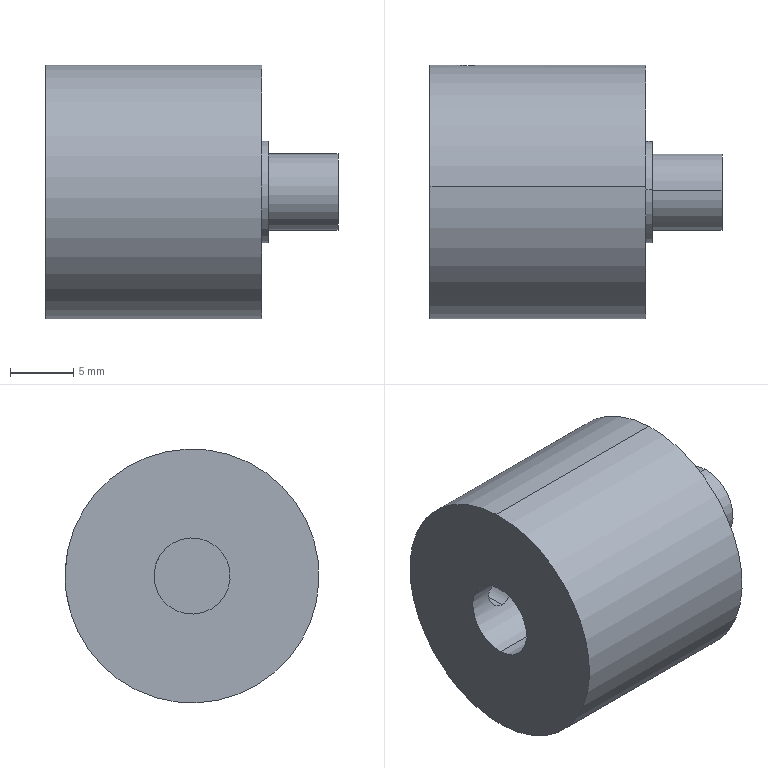Component | SolidWorks | AS-011-JG0108-1 | 1 solid | 15 faces | box 23 x 20 x 20 mm | volume 5133 mm3 | cylinder 10 | plane 5 | commonest cylinder face diameters 6 x4 2.5 x2 20 x2 8 x2
build123d program:
from build123d import *

# Parameters (mm, degrees)
SKETCH2_R          = 1.25
CUT_EXTRUDE1_DEPTH = 22
CUT_EXTRUDE2_START = -36
SKETCH3_R          = 15
SKETCH3_R_2        = 10
CUT_EXTRUDE2_DEPTH = 36


with BuildPart() as part:
    # Sketch1 → Revolve1 (revolve)
    with BuildSketch(Plane.XY, mode=Mode.PRIVATE) as revolve1_sk:
        Polygon((-6, 15), (-23, 15), (-23, 3), (-10.5, 3), (-10.5, 0), (0, 0), (0, 3), (-5.5, 3), (-5.5, 4), (-6, 4), align=None)
    revolve(revolve1_sk.sketch.rotate(Axis((-10.5, 0, 0), (1, 0, 0)), 90), axis=Axis((-10.5, 0, 0), (1, 0, 0)))

    # Sketch2 → Cut-Extrude1 (cut)
    with BuildSketch(Plane(origin=(0, 0, 0), x_dir=(1, 0, 0), z_dir=(0, 1, 0))):
        with Locations(Location((-20, 0, 0), (0, 0, 270))):
            Circle(SKETCH2_R)
    extrude(amount=-CUT_EXTRUDE1_DEPTH, mode=Mode.SUBTRACT)

    # Sketch3 → Cut-Extrude2 (cut)
    with BuildSketch(Plane(origin=(-6, 0, 0), x_dir=(0, 0, -1), z_dir=(1, 0, 0)).offset(CUT_EXTRUDE2_START)):
        Circle(SKETCH3_R)
        Circle(SKETCH3_R_2, mode=Mode.SUBTRACT)
    extrude(amount=CUT_EXTRUDE2_DEPTH, mode=Mode.SUBTRACT)


solid = part.part

# Placed as in the assembly
solid = solid.moved(Location((-0.5, -18, -10), (177.746, 0, 0.001754)))
STEP:
#1=CARTESIAN_POINT('',(-0.8071,-0.3164,-0.3598));
#2=VERTEX_POINT('',#1);
#3=CARTESIAN_POINT('',(-0.8071,-0.3203,-0.4582));
#4=VERTEX_POINT('',#3);
#5=CARTESIAN_POINT('',(-0.8071,-0.3164,-0.3598));
#6=CARTESIAN_POINT('',(-0.8135,-0.3164,-0.3598));
#7=CARTESIAN_POINT('',(-0.82,-0.3163,-0.3611));
#8=CARTESIAN_POINT('',(-0.8318,-0.3159,-0.366));
#9=CARTESIAN_POINT('',(-0.8373,-0.3157,-0.3697));
#10=CARTESIAN_POINT('',(-0.8464,-0.3152,-0.3788));
#11=CARTESIAN_POINT('',(-0.8501,-0.315,-0.3843));
#12=CARTESIAN_POINT('',(-0.855,-0.3149,-0.3962));
#13=CARTESIAN_POINT('',(-0.8563,-0.315,-0.4026));
#14=CARTESIAN_POINT('',(-0.8563,-0.3155,-0.4156));
#15=CARTESIAN_POINT('',(-0.855,-0.3159,-0.422));
#16=CARTESIAN_POINT('',(-0.8501,-0.317,-0.4338));
#17=CARTESIAN_POINT('',(-0.8464,-0.3176,-0.4393));
#18=CARTESIAN_POINT('',(-0.8374,-0.3187,-0.4483));
#19=CARTESIAN_POINT('',(-0.8319,-0.3193,-0.452));
#20=CARTESIAN_POINT('',(-0.8201,-0.3201,-0.4569));
#21=CARTESIAN_POINT('',(-0.8136,-0.3203,-0.4582));
#22=CARTESIAN_POINT('',(-0.8071,-0.3203,-0.4582));
#23=B_SPLINE_CURVE_WITH_KNOTS('',3,(#5,#6,#7,#8,#9,#10,#11,#12,#13,#14,#15,#16,#17,#18,#19,#20,#21,#22),.UNSPECIFIED.,.F.,.F.,(4,2,2,2,2,2,2,2,4),(0.003912,0.004401,0.00489,0.005379,0.005867,0.006356,0.006845,0.007334,0.007823),.UNSPECIFIED.);
#24=EDGE_CURVE('',#2,#4,#23,.T.);
#25=ORIENTED_EDGE('',*,*,#24,.F.);
#26=CARTESIAN_POINT('',(-0.8071,-0.5994,-0.3487));
#27=VERTEX_POINT('',#26);
#28=CARTESIAN_POINT('',(-0.8071,0.1587,-0.3784));
#29=DIRECTION('',(0.,-0.9992,0.03916));
#30=VECTOR('',#29,39.37);
#31=LINE('',#28,#30);
#32=EDGE_CURVE('',#2,#27,#31,.T.);
#33=ORIENTED_EDGE('',*,*,#32,.T.);
#34=CARTESIAN_POINT('',(-0.8071,-0.6033,-0.4471));
#35=VERTEX_POINT('',#34);
#36=CARTESIAN_POINT('',(-0.8071,-0.6033,-0.4471));
#37=CARTESIAN_POINT('',(-0.8104,-0.6033,-0.4471));
#38=CARTESIAN_POINT('',(-0.8136,-0.6031,-0.4468));
#39=CARTESIAN_POINT('',(-0.8199,-0.6025,-0.4455));
#40=CARTESIAN_POINT('',(-0.8231,-0.6021,-0.4446));
#41=CARTESIAN_POINT('',(-0.832,-0.6004,-0.4409));
#42=CARTESIAN_POINT('',(-0.8374,-0.5988,-0.4373));
#43=CARTESIAN_POINT('',(-0.8464,-0.5957,-0.4285));
#44=CARTESIAN_POINT('',(-0.85,-0.5941,-0.4231));
#45=CARTESIAN_POINT('',(-0.855,-0.5917,-0.4114));
#46=CARTESIAN_POINT('',(-0.8563,-0.5909,-0.4049));
#47=CARTESIAN_POINT('',(-0.8563,-0.5905,-0.3951));
#48=CARTESIAN_POINT('',(-0.856,-0.5905,-0.3918));
#49=CARTESIAN_POINT('',(-0.8547,-0.5908,-0.3854));
#50=CARTESIAN_POINT('',(-0.8537,-0.5911,-0.3823));
#51=CARTESIAN_POINT('',(-0.85,-0.5922,-0.3733));
#52=CARTESIAN_POINT('',(-0.8464,-0.5933,-0.3679));
#53=CARTESIAN_POINT('',(-0.8373,-0.5957,-0.3588));
#54=CARTESIAN_POINT('',(-0.8319,-0.597,-0.3551));
#55=CARTESIAN_POINT('',(-0.8201,-0.5989,-0.3501));
#56=CARTESIAN_POINT('',(-0.8136,-0.5994,-0.3487));
#57=CARTESIAN_POINT('',(-0.8071,-0.5994,-0.3487));
#58=B_SPLINE_CURVE_WITH_KNOTS('',3,(#36,#37,#38,#39,#40,#41,#42,#43,#44,#45,#46,#47,#48,#49,#50,#51,#52,#53,#54,#55,#56,#57),.UNSPECIFIED.,.F.,.F.,(4,2,2,2,2,2,2,2,2,2,4),(0.,0.0002471,0.0004942,0.0009884,0.001483,0.001977,0.002224,0.002471,0.002965,0.003459,0.003953),.UNSPECIFIED.);
#59=EDGE_CURVE('',#35,#27,#58,.T.);
#60=ORIENTED_EDGE('',*,*,#59,.F.);
#61=CARTESIAN_POINT('',(-0.8071,0.1549,-0.4768));
#62=DIRECTION('',(0.,-0.9992,0.03916));
#63=VECTOR('',#62,39.37);
#64=LINE('',#61,#63);
#65=EDGE_CURVE('',#4,#35,#64,.T.);
#66=ORIENTED_EDGE('',*,*,#65,.F.);
#67=EDGE_LOOP('',(#25,#33,#60,#66));
#68=FACE_OUTER_BOUND('',#67,.T.);
#69=CARTESIAN_POINT('',(-0.8071,0.1568,-0.4276));
#70=DIRECTION('',(0.,-0.9992,0.03916));
#71=DIRECTION('',(0.,-0.03916,-0.9992));
#72=AXIS2_PLACEMENT_3D('',#69,#70,#71);
#73=CYLINDRICAL_SURFACE('',#72,0.04921);
#74=ADVANCED_FACE('',(#68),#73,.F.);
#75=ORIENTED_EDGE('',*,*,#59,.T.);
#76=CARTESIAN_POINT('',(-0.8071,-0.5994,-0.3487));
#77=CARTESIAN_POINT('',(-0.8006,-0.5994,-0.3487));
#78=CARTESIAN_POINT('',(-0.7941,-0.5989,-0.3501));
#79=CARTESIAN_POINT('',(-0.7822,-0.597,-0.3551));
#80=CARTESIAN_POINT('',(-0.7768,-0.5957,-0.3588));
#81=CARTESIAN_POINT('',(-0.77,-0.5939,-0.3656));
#82=CARTESIAN_POINT('',(-0.768,-0.5933,-0.3681));
#83=CARTESIAN_POINT('',(-0.7645,-0.5923,-0.3735));
#84=CARTESIAN_POINT('',(-0.7629,-0.5918,-0.3763));
#85=CARTESIAN_POINT('',(-0.7604,-0.5911,-0.3823));
#86=CARTESIAN_POINT('',(-0.7595,-0.5908,-0.3854));
#87=CARTESIAN_POINT('',(-0.7582,-0.5905,-0.3918));
#88=CARTESIAN_POINT('',(-0.7579,-0.5905,-0.3951));
#89=CARTESIAN_POINT('',(-0.7579,-0.5909,-0.4048));
#90=CARTESIAN_POINT('',(-0.7592,-0.5917,-0.4113));
#91=CARTESIAN_POINT('',(-0.7641,-0.5941,-0.4231));
#92=CARTESIAN_POINT('',(-0.7678,-0.5957,-0.4284));
#93=CARTESIAN_POINT('',(-0.7768,-0.5988,-0.4374));
#94=CARTESIAN_POINT('',(-0.7821,-0.6004,-0.4409));
#95=CARTESIAN_POINT('',(-0.7941,-0.6026,-0.4458));
#96=CARTESIAN_POINT('',(-0.8005,-0.6033,-0.4471));
#97=CARTESIAN_POINT('',(-0.8071,-0.6033,-0.4471));
#98=B_SPLINE_CURVE_WITH_KNOTS('',3,(#76,#77,#78,#79,#80,#81,#82,#83,#84,#85,#86,#87,#88,#89,#90,#91,#92,#93,#94,#95,#96,#97),.UNSPECIFIED.,.F.,.F.,(4,2,2,2,2,2,2,2,2,2,4),(0.003953,0.004447,0.004941,0.005188,0.005435,0.005682,0.005929,0.006422,0.006916,0.00741,0.007904),.UNSPECIFIED.);
#99=EDGE_CURVE('',#27,#35,#98,.T.);
#100=ORIENTED_EDGE('',*,*,#99,.T.);
#101=EDGE_LOOP('',(#75,#100));
#102=FACE_BOUND('',#101,.T.);
#103=CARTESIAN_POINT('',(-0.4331,-0.704,-0.2757));
#104=VERTEX_POINT('',#103);
#105=CARTESIAN_POINT('',(-0.4331,-0.7133,-0.5117));
#106=VERTEX_POINT('',#105);
#107=CARTESIAN_POINT('',(-0.4331,-0.7087,-0.3937));
#108=DIRECTION('',(-1.,0.,0.));
#109=DIRECTION('',(0.,-0.03916,-0.9992));
#110=AXIS2_PLACEMENT_3D('',#107,#108,#109);
#111=CIRCLE('',#110,0.1181);
#112=EDGE_CURVE('',#104,#106,#111,.T.);
#113=ORIENTED_EDGE('',*,*,#112,.F.);
#114=CARTESIAN_POINT('',(-0.9252,-0.704,-0.2757));
#115=VERTEX_POINT('',#114);
#116=CARTESIAN_POINT('',(-0.4331,-0.704,-0.2757));
#117=DIRECTION('',(-1.,0.,0.));
#118=VECTOR('',#117,39.37);
#119=LINE('',#116,#118);
#120=EDGE_CURVE('',#104,#115,#119,.T.);
#121=ORIENTED_EDGE('',*,*,#120,.T.);
#122=CARTESIAN_POINT('',(-0.9252,-0.7133,-0.5117));
#123=VERTEX_POINT('',#122);
#124=CARTESIAN_POINT('',(-0.9252,-0.7087,-0.3937));
#125=DIRECTION('',(-1.,0.,0.));
#126=DIRECTION('',(0.,-0.03916,-0.9992));
#127=AXIS2_PLACEMENT_3D('',#124,#125,#126);
#128=CIRCLE('',#127,0.1181);
#129=EDGE_CURVE('',#115,#123,#128,.T.);
#130=ORIENTED_EDGE('',*,*,#129,.T.);
#131=CARTESIAN_POINT('',(-0.4331,-0.7133,-0.5117));
#132=DIRECTION('',(-1.,0.,0.));
#133=VECTOR('',#132,39.37);
#134=LINE('',#131,#133);
#135=EDGE_CURVE('',#106,#123,#134,.T.);
#136=ORIENTED_EDGE('',*,*,#135,.F.);
#137=EDGE_LOOP('',(#113,#121,#130,#136));
#138=FACE_OUTER_BOUND('',#137,.T.);
#139=CARTESIAN_POINT('',(-0.4331,-0.7087,-0.3937));
#140=DIRECTION('',(-1.,0.,0.));
#141=DIRECTION('',(0.,-0.03916,-0.9992));
#142=AXIS2_PLACEMENT_3D('',#139,#140,#141);
#143=CYLINDRICAL_SURFACE('',#142,0.1181);
#144=ADVANCED_FACE('',(#102,#138),#143,.F.);
#145=CARTESIAN_POINT('',(-0.9252,-0.6932,-0.000302));
#146=VERTEX_POINT('',#145);
#147=CARTESIAN_POINT('',(-0.9252,-0.7241,-0.7871));
#148=VERTEX_POINT('',#147);
#149=CARTESIAN_POINT('',(-0.9252,-0.7087,-0.3937));
#150=DIRECTION('',(1.,0.,0.));
#151=DIRECTION('',(0.,0.03916,0.9992));
#152=AXIS2_PLACEMENT_3D('',#149,#150,#151);
#153=CIRCLE('',#152,0.3937);
#154=EDGE_CURVE('',#146,#148,#153,.T.);
#155=ORIENTED_EDGE('',*,*,#154,.T.);
#156=CARTESIAN_POINT('',(-0.2559,-0.7241,-0.7871));
#157=VERTEX_POINT('',#156);
#158=CARTESIAN_POINT('',(-1.673,-0.7241,-0.7871));
#159=DIRECTION('',(1.,0.,0.));
#160=VECTOR('',#159,39.37);
#161=LINE('',#158,#160);
#162=EDGE_CURVE('',#148,#157,#161,.T.);
#163=ORIENTED_EDGE('',*,*,#162,.T.);
#164=CARTESIAN_POINT('',(-0.2559,-0.6932,-0.000302));
#165=VERTEX_POINT('',#164);
#166=CARTESIAN_POINT('',(-0.2559,-0.7087,-0.3937));
#167=DIRECTION('',(1.,0.,0.));
#168=DIRECTION('',(0.,0.03916,0.9992));
#169=AXIS2_PLACEMENT_3D('',#166,#167,#168);
#170=CIRCLE('',#169,0.3937);
#171=EDGE_CURVE('',#165,#157,#170,.T.);
#172=ORIENTED_EDGE('',*,*,#171,.F.);
#173=CARTESIAN_POINT('',(-1.673,-0.6932,-0.000302));
#174=DIRECTION('',(1.,0.,0.));
#175=VECTOR('',#174,39.37);
#176=LINE('',#173,#175);
#177=EDGE_CURVE('',#146,#165,#176,.T.);
#178=ORIENTED_EDGE('',*,*,#177,.F.);
#179=EDGE_LOOP('',(#155,#163,#172,#178));
#180=FACE_OUTER_BOUND('',#179,.T.);
#181=CARTESIAN_POINT('',(-1.673,-0.7087,-0.3937));
#182=DIRECTION('',(1.,0.,0.));
#183=DIRECTION('',(0.,0.03916,0.9992));
#184=AXIS2_PLACEMENT_3D('',#181,#182,#183);
#185=CYLINDRICAL_SURFACE('',#184,0.3937);
#186=ADVANCED_FACE('',(#180),#185,.T.);
#187=CARTESIAN_POINT('',(-0.01969,-0.7133,-0.5117));
#188=VERTEX_POINT('',#187);
#189=CARTESIAN_POINT('',(-0.01969,-0.704,-0.2757));
#190=VERTEX_POINT('',#189);
#191=CARTESIAN_POINT('',(-0.01969,-0.7087,-0.3937));
#192=DIRECTION('',(-1.,0.,0.));
#193=DIRECTION('',(0.,-0.03916,-0.9992));
#194=AXIS2_PLACEMENT_3D('',#191,#192,#193);
#195=CIRCLE('',#194,0.1181);
#196=EDGE_CURVE('',#188,#190,#195,.T.);
#197=ORIENTED_EDGE('',*,*,#196,.T.);
#198=CARTESIAN_POINT('',(-0.2362,-0.704,-0.2757));
#199=VERTEX_POINT('',#198);
#200=CARTESIAN_POINT('',(-0.4331,-0.704,-0.2757));
#201=DIRECTION('',(-1.,0.,0.));
#202=VECTOR('',#201,39.37);
#203=LINE('',#200,#202);
#204=EDGE_CURVE('',#190,#199,#203,.T.);
#205=ORIENTED_EDGE('',*,*,#204,.T.);
#206=CARTESIAN_POINT('',(-0.2362,-0.7133,-0.5117));
#207=VERTEX_POINT('',#206);
#208=CARTESIAN_POINT('',(-0.2362,-0.7087,-0.3937));
#209=DIRECTION('',(-1.,0.,0.));
#210=DIRECTION('',(0.,-0.03916,-0.9992));
#211=AXIS2_PLACEMENT_3D('',#208,#209,#210);
#212=CIRCLE('',#211,0.1181);
#213=EDGE_CURVE('',#207,#199,#212,.T.);
#214=ORIENTED_EDGE('',*,*,#213,.F.);
#215=CARTESIAN_POINT('',(-0.4331,-0.7133,-0.5117));
#216=DIRECTION('',(-1.,0.,0.));
#217=VECTOR('',#216,39.37);
#218=LINE('',#215,#217);
#219=EDGE_CURVE('',#188,#207,#218,.T.);
#220=ORIENTED_EDGE('',*,*,#219,.F.);
#221=EDGE_LOOP('',(#197,#205,#214,#220));
#222=FACE_OUTER_BOUND('',#221,.T.);
#223=CARTESIAN_POINT('',(-0.4331,-0.7087,-0.3937));
#224=DIRECTION('',(-1.,0.,0.));
#225=DIRECTION('',(0.,-0.03916,-0.9992));
#226=AXIS2_PLACEMENT_3D('',#223,#224,#225);
#227=CYLINDRICAL_SURFACE('',#226,0.1181);
#228=ADVANCED_FACE('',(#222),#227,.T.);
#229=CARTESIAN_POINT('',(-0.2362,-0.7148,-0.5511));
#230=VERTEX_POINT('',#229);
#231=CARTESIAN_POINT('',(-0.2362,-0.7025,-0.2363));
#232=VERTEX_POINT('',#231);
#233=CARTESIAN_POINT('',(-0.2362,-0.7087,-0.3937));
#234=DIRECTION('',(-1.,0.,0.));
#235=DIRECTION('',(0.,-0.03916,-0.9992));
#236=AXIS2_PLACEMENT_3D('',#233,#234,#235);
#237=CIRCLE('',#236,0.1575);
#238=EDGE_CURVE('',#230,#232,#237,.T.);
#239=ORIENTED_EDGE('',*,*,#238,.T.);
#240=CARTESIAN_POINT('',(-0.2559,-0.7025,-0.2363));
#241=VERTEX_POINT('',#240);
#242=CARTESIAN_POINT('',(-0.4331,-0.7025,-0.2363));
#243=DIRECTION('',(-1.,0.,0.));
#244=VECTOR('',#243,39.37);
#245=LINE('',#242,#244);
#246=EDGE_CURVE('',#232,#241,#245,.T.);
#247=ORIENTED_EDGE('',*,*,#246,.T.);
#248=CARTESIAN_POINT('',(-0.2559,-0.7148,-0.5511));
#249=VERTEX_POINT('',#248);
#250=CARTESIAN_POINT('',(-0.2559,-0.7087,-0.3937));
#251=DIRECTION('',(-1.,0.,0.));
#252=DIRECTION('',(0.,-0.03916,-0.9992));
#253=AXIS2_PLACEMENT_3D('',#250,#251,#252);
#254=CIRCLE('',#253,0.1575);
#255=EDGE_CURVE('',#249,#241,#254,.T.);
#256=ORIENTED_EDGE('',*,*,#255,.F.);
#257=CARTESIAN_POINT('',(-0.4331,-0.7148,-0.5511));
#258=DIRECTION('',(-1.,0.,0.));
#259=VECTOR('',#258,39.37);
#260=LINE('',#257,#259);
#261=EDGE_CURVE('',#230,#249,#260,.T.);
#262=ORIENTED_EDGE('',*,*,#261,.F.);
#263=EDGE_LOOP('',(#239,#247,#256,#262));
#264=FACE_OUTER_BOUND('',#263,.T.);
#265=CARTESIAN_POINT('',(-0.4331,-0.7087,-0.3937));
#266=DIRECTION('',(-1.,0.,0.));
#267=DIRECTION('',(0.,-0.03916,-0.9992));
#268=AXIS2_PLACEMENT_3D('',#265,#266,#267);
#269=CYLINDRICAL_SURFACE('',#268,0.1575);
#270=ADVANCED_FACE('',(#264),#269,.T.);
#271=ORIENTED_EDGE('',*,*,#255,.T.);
#272=CARTESIAN_POINT('',(-0.2559,-0.7087,-0.3937));
#273=DIRECTION('',(-1.,0.,0.));
#274=DIRECTION('',(0.,-0.03916,-0.9992));
#275=AXIS2_PLACEMENT_3D('',#272,#273,#274);
#276=CIRCLE('',#275,0.1575);
#277=EDGE_CURVE('',#241,#249,#276,.T.);
#278=ORIENTED_EDGE('',*,*,#277,.T.);
#279=EDGE_LOOP('',(#271,#278));
#280=FACE_BOUND('',#279,.T.);
#281=ORIENTED_EDGE('',*,*,#171,.T.);
#282=CARTESIAN_POINT('',(-0.2559,-0.7087,-0.3937));
#283=DIRECTION('',(1.,0.,0.));
#284=DIRECTION('',(0.,0.03916,0.9992));
#285=AXIS2_PLACEMENT_3D('',#282,#283,#284);
#286=CIRCLE('',#285,0.3937);
#287=EDGE_CURVE('',#157,#165,#286,.T.);
#288=ORIENTED_EDGE('',*,*,#287,.T.);
#289=EDGE_LOOP('',(#281,#288));
#290=FACE_OUTER_BOUND('',#289,.T.);
#291=CARTESIAN_POINT('',(-0.2559,-1.299,-0.3706));
#292=DIRECTION('',(-1.,0.,0.));
#293=DIRECTION('',(0.,-0.03916,-0.9992));
#294=AXIS2_PLACEMENT_3D('',#291,#292,#293);
#295=PLANE('',#294);
#296=ADVANCED_FACE('',(#280,#290),#295,.F.);
#297=ORIENTED_EDGE('',*,*,#246,.F.);
#298=CARTESIAN_POINT('',(-0.2362,-0.7087,-0.3937));
#299=DIRECTION('',(-1.,0.,0.));
#300=DIRECTION('',(0.,-0.03916,-0.9992));
#301=AXIS2_PLACEMENT_3D('',#298,#299,#300);
#302=CIRCLE('',#301,0.1575);
#303=EDGE_CURVE('',#232,#230,#302,.T.);
#304=ORIENTED_EDGE('',*,*,#303,.T.);
#305=ORIENTED_EDGE('',*,*,#261,.T.);
#306=ORIENTED_EDGE('',*,*,#277,.F.);
#307=EDGE_LOOP('',(#297,#304,#305,#306));
#308=FACE_OUTER_BOUND('',#307,.T.);
#309=CARTESIAN_POINT('',(-0.4331,-0.7087,-0.3937));
#310=DIRECTION('',(-1.,0.,0.));
#311=DIRECTION('',(0.,-0.03916,-0.9992));
#312=AXIS2_PLACEMENT_3D('',#309,#310,#311);
#313=CYLINDRICAL_SURFACE('',#312,0.1575);
#314=ADVANCED_FACE('',(#308),#313,.T.);
#315=ORIENTED_EDGE('',*,*,#238,.F.);
#316=ORIENTED_EDGE('',*,*,#303,.F.);
#317=EDGE_LOOP('',(#315,#316));
#318=FACE_OUTER_BOUND('',#317,.T.);
#319=ORIENTED_EDGE('',*,*,#213,.T.);
#320=CARTESIAN_POINT('',(-0.2362,-0.7087,-0.3937));
#321=DIRECTION('',(-1.,0.,0.));
#322=DIRECTION('',(0.,-0.03916,-0.9992));
#323=AXIS2_PLACEMENT_3D('',#320,#321,#322);
#324=CIRCLE('',#323,0.1181);
#325=EDGE_CURVE('',#199,#207,#324,.T.);
#326=ORIENTED_EDGE('',*,*,#325,.T.);
#327=EDGE_LOOP('',(#319,#326));
#328=FACE_BOUND('',#327,.T.);
#329=CARTESIAN_POINT('',(-0.2362,-0.866,-0.3875));
#330=DIRECTION('',(-1.,0.,0.));
#331=DIRECTION('',(0.,-0.03916,-0.9992));
#332=AXIS2_PLACEMENT_3D('',#329,#330,#331);
#333=PLANE('',#332);
#334=ADVANCED_FACE('',(#318,#328),#333,.F.);
#335=ORIENTED_EDGE('',*,*,#204,.F.);
#336=CARTESIAN_POINT('',(-0.01969,-0.7087,-0.3937));
#337=DIRECTION('',(-1.,0.,0.));
#338=DIRECTION('',(0.,-0.03916,-0.9992));
#339=AXIS2_PLACEMENT_3D('',#336,#337,#338);
#340=CIRCLE('',#339,0.1181);
#341=EDGE_CURVE('',#190,#188,#340,.T.);
#342=ORIENTED_EDGE('',*,*,#341,.T.);
#343=ORIENTED_EDGE('',*,*,#219,.T.);
#344=ORIENTED_EDGE('',*,*,#325,.F.);
#345=EDGE_LOOP('',(#335,#342,#343,#344));
#346=FACE_OUTER_BOUND('',#345,.T.);
#347=CARTESIAN_POINT('',(-0.4331,-0.7087,-0.3937));
#348=DIRECTION('',(-1.,0.,0.));
#349=DIRECTION('',(0.,-0.03916,-0.9992));
#350=AXIS2_PLACEMENT_3D('',#347,#348,#349);
#351=CYLINDRICAL_SURFACE('',#350,0.1181);
#352=ADVANCED_FACE('',(#346),#351,.T.);
#353=ORIENTED_EDGE('',*,*,#196,.F.);
#354=ORIENTED_EDGE('',*,*,#341,.F.);
#355=EDGE_LOOP('',(#353,#354));
#356=FACE_OUTER_BOUND('',#355,.T.);
#357=CARTESIAN_POINT('',(-0.01969,-0.8267,-0.3891));
#358=DIRECTION('',(-1.,0.,0.));
#359=DIRECTION('',(0.,-0.03916,-0.9992));
#360=AXIS2_PLACEMENT_3D('',#357,#358,#359);
#361=PLANE('',#360);
#362=ADVANCED_FACE('',(#356),#361,.F.);
#363=ORIENTED_EDGE('',*,*,#162,.F.);
#364=CARTESIAN_POINT('',(-0.9252,-0.7087,-0.3937));
#365=DIRECTION('',(1.,0.,0.));
#366=DIRECTION('',(0.,0.03916,0.9992));
#367=AXIS2_PLACEMENT_3D('',#364,#365,#366);
#368=CIRCLE('',#367,0.3937);
#369=EDGE_CURVE('',#148,#146,#368,.T.);
#370=ORIENTED_EDGE('',*,*,#369,.T.);
#371=ORIENTED_EDGE('',*,*,#177,.T.);
#372=ORIENTED_EDGE('',*,*,#287,.F.);
#373=EDGE_LOOP('',(#363,#370,#371,#372));
#374=FACE_OUTER_BOUND('',#373,.T.);
#375=CARTESIAN_POINT('',(-0.8071,-0.3203,-0.4582));
#376=CARTESIAN_POINT('',(-0.8006,-0.3203,-0.4582));
#377=CARTESIAN_POINT('',(-0.7942,-0.3201,-0.4569));
#378=CARTESIAN_POINT('',(-0.7823,-0.3193,-0.452));
#379=CARTESIAN_POINT('',(-0.7768,-0.3187,-0.4483));
#380=CARTESIAN_POINT('',(-0.7677,-0.3176,-0.4393));
#381=CARTESIAN_POINT('',(-0.7641,-0.317,-0.4338));
#382=CARTESIAN_POINT('',(-0.7592,-0.3159,-0.422));
#383=CARTESIAN_POINT('',(-0.7579,-0.3155,-0.4156));
#384=CARTESIAN_POINT('',(-0.7579,-0.3151,-0.4059));
#385=CARTESIAN_POINT('',(-0.7582,-0.315,-0.4027));
#386=CARTESIAN_POINT('',(-0.7595,-0.315,-0.3963));
#387=CARTESIAN_POINT('',(-0.7604,-0.3149,-0.3933));
#388=CARTESIAN_POINT('',(-0.7641,-0.315,-0.3843));
#389=CARTESIAN_POINT('',(-0.7677,-0.3152,-0.3789));
#390=CARTESIAN_POINT('',(-0.7769,-0.3157,-0.3697));
#391=CARTESIAN_POINT('',(-0.7823,-0.3159,-0.3661));
#392=CARTESIAN_POINT('',(-0.7912,-0.3162,-0.3623));
#393=CARTESIAN_POINT('',(-0.7943,-0.3163,-0.3614));
#394=CARTESIAN_POINT('',(-0.8006,-0.3164,-0.3601));
#395=CARTESIAN_POINT('',(-0.8039,-0.3164,-0.3598));
#396=CARTESIAN_POINT('',(-0.8071,-0.3164,-0.3598));
#397=B_SPLINE_CURVE_WITH_KNOTS('',3,(#375,#376,#377,#378,#379,#380,#381,#382,#383,#384,#385,#386,#387,#388,#389,#390,#391,#392,#393,#394,#395,#396),.UNSPECIFIED.,.F.,.F.,(4,2,2,2,2,2,2,2,2,2,4),(0.,0.000489,0.000978,0.001467,0.001956,0.0022,0.002445,0.002934,0.003423,0.003667,0.003912),.UNSPECIFIED.);
#398=EDGE_CURVE('',#4,#2,#397,.T.);
#399=ORIENTED_EDGE('',*,*,#398,.T.);
#400=ORIENTED_EDGE('',*,*,#24,.T.);
#401=EDGE_LOOP('',(#399,#400));
#402=FACE_BOUND('',#401,.T.);
#403=CARTESIAN_POINT('',(-1.673,-0.7087,-0.3937));
#404=DIRECTION('',(1.,0.,0.));
#405=DIRECTION('',(0.,0.03916,0.9992));
#406=AXIS2_PLACEMENT_3D('',#403,#404,#405);
#407=CYLINDRICAL_SURFACE('',#406,0.3937);
#408=ADVANCED_FACE('',(#374,#402),#407,.T.);
#409=CARTESIAN_POINT('',(-0.4331,-0.7087,-0.3937));
#410=DIRECTION('',(-1.,0.,0.));
#411=DIRECTION('',(0.,-0.03916,-0.9992));
#412=AXIS2_PLACEMENT_3D('',#409,#410,#411);
#413=CIRCLE('',#412,0.1181);
#414=EDGE_CURVE('',#106,#104,#413,.T.);
#415=ORIENTED_EDGE('',*,*,#414,.T.);
#416=ORIENTED_EDGE('',*,*,#112,.T.);
#417=EDGE_LOOP('',(#415,#416));
#418=FACE_OUTER_BOUND('',#417,.T.);
#419=CARTESIAN_POINT('',(-0.4331,-0.8267,-0.3891));
#420=DIRECTION('',(1.,0.,0.));
#421=DIRECTION('',(0.,0.03916,0.9992));
#422=AXIS2_PLACEMENT_3D('',#419,#420,#421);
#423=PLANE('',#422);
#424=ADVANCED_FACE('',(#418),#423,.F.);
#425=CARTESIAN_POINT('',(-0.9252,-0.7087,-0.3937));
#426=DIRECTION('',(-1.,0.,0.));
#427=DIRECTION('',(0.,-0.03916,-0.9992));
#428=AXIS2_PLACEMENT_3D('',#425,#426,#427);
#429=CIRCLE('',#428,0.1181);
#430=EDGE_CURVE('',#123,#115,#429,.T.);
#431=ORIENTED_EDGE('',*,*,#430,.F.);
#432=ORIENTED_EDGE('',*,*,#129,.F.);
#433=EDGE_LOOP('',(#431,#432));
#434=FACE_BOUND('',#433,.T.);
#435=ORIENTED_EDGE('',*,*,#154,.F.);
#436=ORIENTED_EDGE('',*,*,#369,.F.);
#437=EDGE_LOOP('',(#435,#436));
#438=FACE_OUTER_BOUND('',#437,.T.);
#439=CARTESIAN_POINT('',(-0.9252,-1.299,-0.3706));
#440=DIRECTION('',(1.,0.,0.));
#441=DIRECTION('',(0.,0.03916,0.9992));
#442=AXIS2_PLACEMENT_3D('',#439,#440,#441);
#443=PLANE('',#442);
#444=ADVANCED_FACE('',(#434,#438),#443,.F.);
#445=ORIENTED_EDGE('',*,*,#120,.F.);
#446=ORIENTED_EDGE('',*,*,#414,.F.);
#447=ORIENTED_EDGE('',*,*,#135,.T.);
#448=ORIENTED_EDGE('',*,*,#430,.T.);
#449=EDGE_LOOP('',(#445,#446,#447,#448));
#450=FACE_OUTER_BOUND('',#449,.T.);
#451=CARTESIAN_POINT('',(-0.4331,-0.7087,-0.3937));
#452=DIRECTION('',(-1.,0.,0.));
#453=DIRECTION('',(0.,-0.03916,-0.9992));
#454=AXIS2_PLACEMENT_3D('',#451,#452,#453);
#455=CYLINDRICAL_SURFACE('',#454,0.1181);
#456=ADVANCED_FACE('',(#450),#455,.F.);
#457=ORIENTED_EDGE('',*,*,#32,.F.);
#458=ORIENTED_EDGE('',*,*,#398,.F.);
#459=ORIENTED_EDGE('',*,*,#65,.T.);
#460=ORIENTED_EDGE('',*,*,#99,.F.);
#461=EDGE_LOOP('',(#457,#458,#459,#460));
#462=FACE_OUTER_BOUND('',#461,.T.);
#463=CARTESIAN_POINT('',(-0.8071,0.1568,-0.4276));
#464=DIRECTION('',(0.,-0.9992,0.03916));
#465=DIRECTION('',(0.,-0.03916,-0.9992));
#466=AXIS2_PLACEMENT_3D('',#463,#464,#465);
#467=CYLINDRICAL_SURFACE('',#466,0.04921);
#468=ADVANCED_FACE('',(#462),#467,.F.);
#469=CLOSED_SHELL('',(#74,#144,#186,#228,#270,#296,#314,#334,#352,#362,#408,#424,#444,#456,#468));
#470=MANIFOLD_SOLID_BREP('',#469);
#471=CARTESIAN_POINT('',(0.,0.,0.));
#472=DIRECTION('',(0.,0.,1.));
#473=DIRECTION('',(1.,0.,0.));
#474=AXIS2_PLACEMENT_3D('',#471,#472,#473);
#475=(LENGTH_UNIT()NAMED_UNIT(*)SI_UNIT($,.METRE.));
#476=LENGTH_MEASURE_WITH_UNIT(LENGTH_MEASURE(0.0254),#475);
#477=DIMENSIONAL_EXPONENTS(1.,0.,0.,0.,0.,0.,0.);
#478=(CONVERSION_BASED_UNIT('',#476)LENGTH_UNIT()NAMED_UNIT(#477));
#479=UNCERTAINTY_MEASURE_WITH_UNIT(LENGTH_MEASURE(0.00001),#478,'','');
#480=(NAMED_UNIT(*)PLANE_ANGLE_UNIT()SI_UNIT($,.RADIAN.));
#481=(NAMED_UNIT(*)SI_UNIT($,.STERADIAN.)SOLID_ANGLE_UNIT());
#482=(GEOMETRIC_REPRESENTATION_CONTEXT(3)GLOBAL_UNCERTAINTY_ASSIGNED_CONTEXT((#479))GLOBAL_UNIT_ASSIGNED_CONTEXT((#478,#480,#481))REPRESENTATION_CONTEXT('',''));
#483=ADVANCED_BREP_SHAPE_REPRESENTATION('',(#470,#474),#482);
#484=COLOUR_RGB('',0.7922,0.8196,0.9333);
#485=FILL_AREA_STYLE_COLOUR('',#484);
#486=FILL_AREA_STYLE('',(#485));
#487=SURFACE_STYLE_FILL_AREA(#486);
#488=SURFACE_SIDE_STYLE('',(#487));
#489=SURFACE_STYLE_USAGE(.BOTH.,#488);
#490=PRESENTATION_STYLE_ASSIGNMENT((#489));
#491=STYLED_ITEM('',(#490),#470);
#492=(LENGTH_UNIT()NAMED_UNIT(*)SI_UNIT($,.METRE.));
#493=LENGTH_MEASURE_WITH_UNIT(LENGTH_MEASURE(0.0254),#492);
#494=DIMENSIONAL_EXPONENTS(1.,0.,0.,0.,0.,0.,0.);
#495=(CONVERSION_BASED_UNIT('',#493)LENGTH_UNIT()NAMED_UNIT(#494));
#496=UNCERTAINTY_MEASURE_WITH_UNIT(LENGTH_MEASURE(0.00001),#495,'','');
#497=(NAMED_UNIT(*)PLANE_ANGLE_UNIT()SI_UNIT($,.RADIAN.));
#498=(NAMED_UNIT(*)SI_UNIT($,.STERADIAN.)SOLID_ANGLE_UNIT());
#499=(GEOMETRIC_REPRESENTATION_CONTEXT(3)GLOBAL_UNCERTAINTY_ASSIGNED_CONTEXT((#496))GLOBAL_UNIT_ASSIGNED_CONTEXT((#495,#497,#498))REPRESENTATION_CONTEXT('',''));
#500=MECHANICAL_DESIGN_GEOMETRIC_PRESENTATION_REPRESENTATION('',(#491),#499);
#501=PRESENTATION_LAYER_ASSIGNMENT('','',(#491));